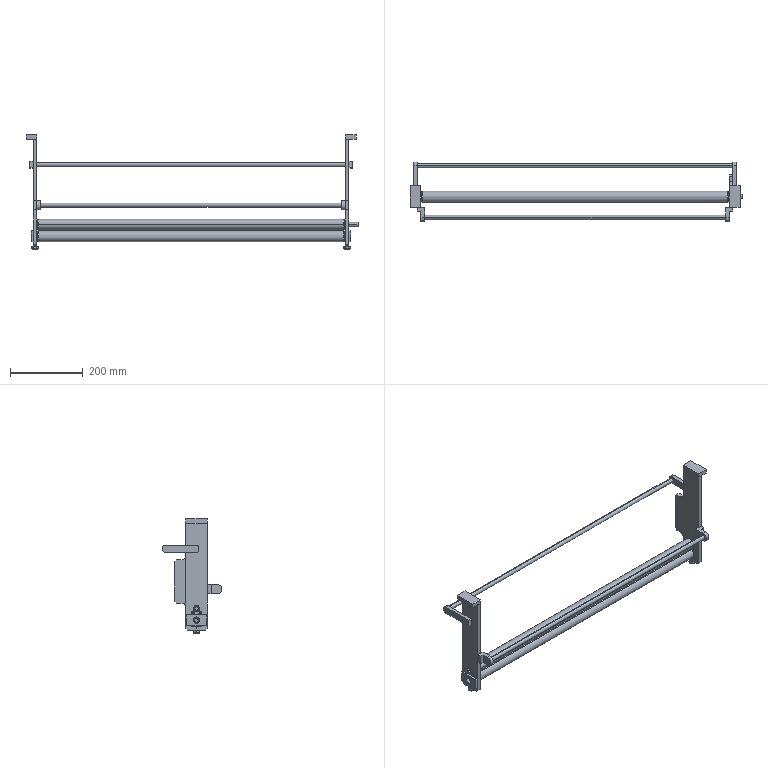Assembly | SolidWorks | mm | 15 component files | 18 solids | 370 faces | box 914 x 165 x 314.4 mm | volume 1892021 mm3 | plane 166 | cylinder 126 | spline 40 | cone 38 | commonest cylinder face diameters 12 x24 8 x20 21 x16 19 x16 14.78 x16 15 x8 18 x8 30 x4
Bill of materials:
hex nuts, style 1-grades ab gb | 2 |  | Hexagonal prismatic body with a central round through-bore and chamfered corners on both faces; hex-nut-like shape.
D012 | 1 |  | Long slender round rod with a flat rectangular tab at each end; the tabs sit perpendicular to the rod and point the same way, giving a U/staple-like outline.
D014 | 1 |  | Long slender round rod ending in a small stepped, hook-like or L-profile block at each end; the end blocks have a rounded (D-shaped) outline.
MainFeedAxis3 | 1 |  | Long cylindrical rod/shaft with a reduced-diameter stub at each end; one stub is very short and the other noticeably longer.
SB6801ZZ_2_14 | 4 |  | Plain annular ring/thick washer: a short cylinder with a large central through-hole and slightly rounded edges.
SupportPlate3 | 1 |  | Thin flat elongated plate with a stepped side profile: a protruding tab with filleted inner corners partway along one edge, plus a round hole and a square/rectangular cutout near one end.
MainFeedAxis1 | 1 |  | Long cylindrical rod with a short reduced-diameter stub at each end; the end view shows a stepped concentric shoulder pattern.
Part2^SW-451 | 1 |  | Two separate, identical small rectangular blocks spaced far apart along one axis, with no visible connecting geometry.
SupportPlate1 | 2 |  | Rectangular block with a stepped (L-shaped) cross-section and a large round through-hole, carrying two helical coil springs that stick out from the top face.
SupportPlate | 1 |  | Thin flat rectangular strip with chamfered corners at one end, a round hole and a rectangular window near that end.
Mates:
1. coincident | DriveAxis-1/SupportPlate3-1 face at (869, -15, -207.268) dir (0, -1, 0) | SupportPlate1-1 face at (859, -15, -189.268) dir (0, 1, 0)
2. concentric | DrivenAxis-1/SB6801ZZ_2_14-1 face at (10, -30, -174.268) dir (-1, 0, 0) r 10.5 | SupportPlate1-2 face at (5, -30, -174.268) dir (1, 0, 0) r 10.5
3. concentric | DriveAxis-1/SB6801ZZ_2_14-2 face at (10, -30, -142.268) dir (-1, 0, 0) r 10.5 | SupportPlate-2 face at (5, -30, -142.268) dir (1, 0, 0) r 10.5
4. coincident | DriveAxis-1/SB6801ZZ_2_14-2 face at (5, -22.521, -149.204) dir (-1, 0, 0) | SupportPlate-2 face at (5, -30, -142.268) dir (1, 0, 0)
5. coincident | SupportPlate1-2 face at (10, -45, -189.268) dir (0, -1, 0) | SupportPlate-2 face at (0, -45, -207.268) dir (0, 1, 0)
6. concentric | DrivenAxis-1/SB6801ZZ_2_14-2 face at (864, -30, -174.268) dir (-1, 0, 0) r 10.5 | SupportPlate1-1 face at (864, -30, -174.268) dir (-1, 0, 0) r 10.5
7. coincident | DrivenAxis-1/SB6801ZZ_2_14-2 face at (864, -26.884, -165.294) dir (1, 0, 0) | SupportPlate1-1 face at (864, -30, -174.268) dir (-1, 0, 0)
8. coincident | DrivenAxis-1/SB6801ZZ_2_14-1 face at (5, -26.655, -164.632) dir (-1, 0, 0) | SupportPlate1-2 face at (5, -30, -174.268) dir (1, 0, 0)
9. coincident | SupportPlate1-2 face at (0, -15, -189.268) dir (1, 0, 0) | SupportPlate-2 face at (0, 0, -207.268) dir (-1, 0, 0)
10. distance | SupportPlate1-2 face at (10, -15, -159.268) dir (0, 0, 1) | SupportPlate-2 face at (0, -15, -157.268) dir (0, 0, -1)
11. concentric | DriveAxis-1/SupportPlate3-1 face at (864, -30, -201.268) dir (0, 0, -1) r 3.4 | assembly face at (864, -30, -190.552) dir (0, 0, 1) r 4
12. coincident | DriveAxis-1/SupportPlate3-1 face at (869, -69.775, -201.268) dir (0, 0, -1) | AdjustmentMechanism-1/hex nuts, style 1-grades ab gb-1 face at (859.368, -22.008, -201.268) dir (0, 0, 1)
13. concentric | SupportPlate-2 face at (5, -30, -201.268) dir (0, 0, -1) r 3.4 | assembly face at (5, -30, -190.552) dir (0, 0, 1) r 4
14. coincident | SupportPlate-2 face at (0, 9.775, -201.268) dir (0, 0, -1) | AdjustmentMechanism-2/hex nuts, style 1-grades ab gb-1 face at (0.07306, -22.186, -201.268) dir (0, 0, 1)
15. coincident | SupportPlate-2 face at (0, 0, -207.268) dir (-1, 0, 0) | assembly plane at (0, 0, 0) dir (1, 0, 0)
16. coincident | SupportPlate-2 face at (10, 0, -207.268) dir (0, 1, 0) | assembly plane at (0, 0, 0) dir (0, 1, 0)
17. width | Part2^SW-451-1 face at (889, -60, 104.732) dir (1, 0, 0) | Part2^SW-451-1 face at (-20, -60, 104.732) dir (-1, 0, 0) | SupportPlate-2 face at (0, 0, -207.268) dir (-1, 0, 0) | DriveAxis-1/SupportPlate3-1 face at (869, -60, -207.268) dir (1, 0, 0)
18. coincident | DriveAxis-1/SupportPlate3-1 face at (859, 0, -207.268) dir (0, 1, 0) | Part2^SW-451-1 face at (-20, 0, 104.732) dir (0, 1, 0)
19. coincident | DriveAxis-1/SupportPlate3-1 face at (859, -60, 92.732) dir (0, 0, 1) | Part2^SW-451-1 face at (-20, -60, 92.732) dir (0, 0, -1)
20. coincident | DriveAxis-1/SupportPlate3-1 face at (869, -60, -207.268) dir (1, 0, 0) | D012-1 face at (869, -35, 32.732) dir (-1, 0, 0)
21. distance | D012-1 face at (869, -35, 32.732) dir (0, -1, 0) | DriveAxis-1/SupportPlate3-1 face at (859, 0, -207.268) dir (0, 1, 0)
22. distance | D012-1 face at (869, -35, 12.732) dir (0, 0, -1) | DriveAxis-1/SupportPlate3-1 face at (859, 30, -7.268) dir (0, 0, 1)
23. perpendicular | DriveAxis-1/SupportPlate3-1 face at (859, -60, -207.268) dir (0, -1, 0) | D014-1 face at (849, -60, -101.268) dir (0, 0, -1)
24. coincident | SupportPlate-2 face at (10, 0, -207.268) dir (1, 0, 0) | D014-1 face at (10, -87.5, -88.768) dir (-1, 0, 0)
25. coincident | DriveAxis-1/SupportPlate3-1 face at (859, -60, -207.268) dir (0, -1, 0) | D014-1 face at (849, -60, -101.268) dir (0, 1, 0)
26. distance | D014-1 face at (849, -60, -101.268) dir (0, 0, -1) | DriveAxis-1/SupportPlate3-1 face at (869, -69.775, -201.268) dir (0, 0, -1)
27. concentric | MainFeedAxis3-1 face at (-9.333, -10.69, 846) dir (0, 0, -1) r 7.5 | SB6801ZZ_2_14-1 face at (-9.333, -10.69, -8) dir (0, 0, 1) r 6
28. coincident | MainFeedAxis3-1 face at (-9.333, -10.69, -3) dir (0, 0, -1) | SB6801ZZ_2_14-1 face at (-3.915, -5.665, -3) dir (0, 0, 1)
29. concentric | MainFeedAxis3-1 face at (-9.333, -10.69, 846) dir (0, 0, -1) r 7.5 | SB6801ZZ_2_14-2 face at (-9.333, -10.69, 846) dir (0, 0, 1) r 6
30. coincident | MainFeedAxis3-1 face at (-9.333, -10.69, 846) dir (0, 0, 1) | SB6801ZZ_2_14-2 face at (-4.714, -6.406, 846) dir (0, 0, -1)
31. concentric | SB6801ZZ_2_14-1 face at (-9.333, -10.69, -8) dir (0, 0, 1) r 10.5 | SupportPlate3-1 face at (-9.333, -10.69, -8) dir (0, 0, 1) r 10.5
32. coincident | SB6801ZZ_2_14-1 face at (-2.368, -4.23, -8) dir (0, 0, -1) | SupportPlate3-1 face at (-9.333, -10.69, -8) dir (0, 0, 1)
33. coincident | MainFeedAxis1-1 edge at (0, 0, 846) dir (0, 0, 1) r 6 | SB6801ZZ_2_14-1 face at (0, 0, 846) dir (0, 0, 1) r 6
34. coincident | MainFeedAxis1-1 face at (0, 0, 846) dir (0, 0, 1) | SB6801ZZ_2_14-1 face at (4.619, 4.284, 846) dir (0, 0, -1)
35. concentric | MainFeedAxis1-1 face at (0, 0, -11) dir (0, 0, 1) r 6 | SB6801ZZ_2_14-2 face at (0, 0, -8) dir (0, 0, 1) r 6
36. coincident | MainFeedAxis1-1 face at (0, 0, -3) dir (0, 0, -1) | SB6801ZZ_2_14-2 face at (5.418, 5.025, -3) dir (0, 0, 1)